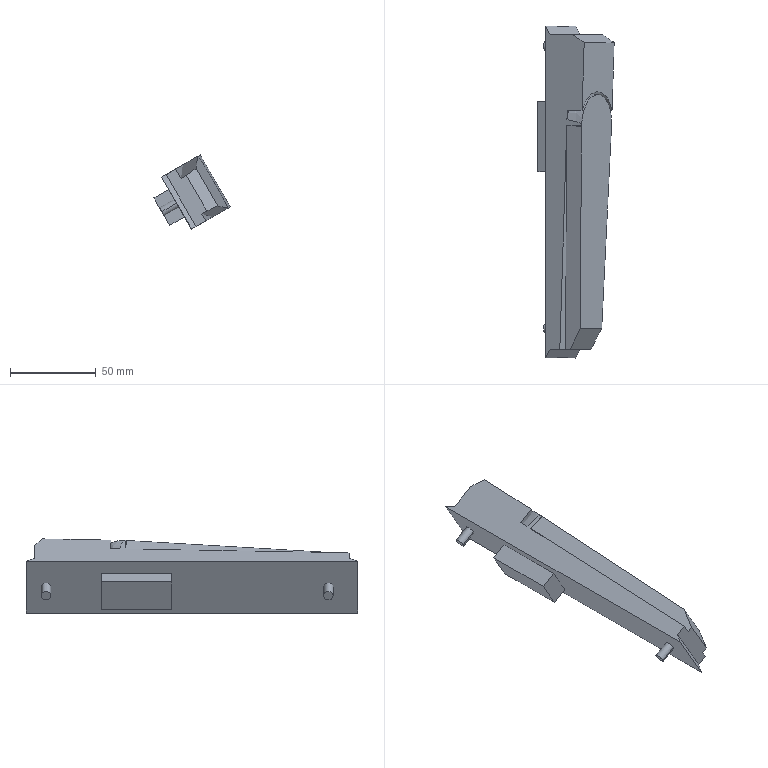Component | SolidWorks | FrontDoorAssembly-1_MS829-1 | 1 solid | 33 faces | box 44.55 x 194 x 43.31 mm | volume 146301 mm3 | plane 24 | cylinder 5 | cone 4 | commonest cylinder face diameters 5.5 x4 35 x1 | material Malleable Cast Iron
STEP:
#1=CARTESIAN_POINT('',(-2.241,37.207,42.755));
#2=VERTEX_POINT('',#1);
#3=CARTESIAN_POINT('',(-2.6,36.76,43.343));
#4=VERTEX_POINT('',#3);
#5=CARTESIAN_POINT('',(-2.265,36.453,42.741));
#6=DIRECTION('',(0.8655,-0.03589,0.4997));
#7=DIRECTION('',(0.03108,0.9994,0.01795));
#8=AXIS2_PLACEMENT_3D('',#5,#6,#7);
#9=CIRCLE('',#8,0.7544);
#10=EDGE_CURVE('',#2,#4,#9,.T.);
#11=ORIENTED_EDGE('',*,*,#10,.F.);
#12=CARTESIAN_POINT('',(-1.9,37.2,42.952));
#13=VERTEX_POINT('',#12);
#14=CARTESIAN_POINT('',(-1.9,37.2,42.952));
#15=DIRECTION('',(0.8659,-0.01845,0.4999));
#16=VECTOR('',#15,39.37);
#17=LINE('',#14,#16);
#18=EDGE_CURVE('',#2,#13,#17,.T.);
#19=ORIENTED_EDGE('',*,*,#18,.T.);
#20=CARTESIAN_POINT('',(-2.258,36.763,43.541));
#21=VERTEX_POINT('',#20);
#22=CARTESIAN_POINT('',(-1.924,36.439,42.938));
#23=DIRECTION('',(0.8655,-0.03589,0.4997));
#24=DIRECTION('',(0.03108,0.9994,0.01795));
#25=AXIS2_PLACEMENT_3D('',#22,#23,#24);
#26=CIRCLE('',#25,0.7613);
#27=EDGE_CURVE('',#13,#21,#26,.T.);
#28=ORIENTED_EDGE('',*,*,#27,.T.);
#29=CARTESIAN_POINT('',(-2.258,36.763,43.541));
#30=CARTESIAN_POINT('',(-2.372,36.762,43.475));
#31=CARTESIAN_POINT('',(-2.486,36.761,43.409));
#32=CARTESIAN_POINT('',(-2.6,36.76,43.343));
#33=B_SPLINE_CURVE_WITH_KNOTS('',3,(#29,#30,#31,#32),.UNSPECIFIED.,.F.,.F.,(4,4),(0.03013,0.04013),.UNSPECIFIED.);
#34=EDGE_CURVE('',#21,#4,#33,.T.);
#35=ORIENTED_EDGE('',*,*,#34,.T.);
#36=EDGE_LOOP('',(#11,#19,#28,#35));
#37=FACE_OUTER_BOUND('',#36,.T.);
#38=CARTESIAN_POINT('',(-1.924,36.439,42.938));
#39=DIRECTION('',(0.8655,-0.03589,0.4997));
#40=DIRECTION('',(0.03108,0.9994,0.01795));
#41=AXIS2_PLACEMENT_3D('',#38,#39,#40);
#42=CONICAL_SURFACE('',#41,0.7613,0.01745);
#43=ADVANCED_FACE('',(#37),#42,.F.);
#44=CARTESIAN_POINT('',(-2.268,36.439,43.535));
#45=VERTEX_POINT('',#44);
#46=CARTESIAN_POINT('',(-1.902,37.128,42.95));
#47=VERTEX_POINT('',#46);
#48=CARTESIAN_POINT('',(-1.924,36.439,42.938));
#49=DIRECTION('',(-0.8655,0.03589,-0.4997));
#50=DIRECTION('',(0.03108,0.9994,0.01795));
#51=AXIS2_PLACEMENT_3D('',#48,#49,#50);
#52=CIRCLE('',#51,0.689);
#53=EDGE_CURVE('',#45,#47,#52,.T.);
#54=ORIENTED_EDGE('',*,*,#53,.T.);
#55=CARTESIAN_POINT('',(-2.243,37.149,42.754));
#56=VERTEX_POINT('',#55);
#57=CARTESIAN_POINT('',(-1.902,37.128,42.95));
#58=DIRECTION('',(-0.8648,0.05333,-0.4993));
#59=VECTOR('',#58,39.37);
#60=LINE('',#57,#59);
#61=EDGE_CURVE('',#47,#56,#60,.T.);
#62=ORIENTED_EDGE('',*,*,#61,.T.);
#63=CARTESIAN_POINT('',(-2.606,36.551,43.34));
#64=VERTEX_POINT('',#63);
#65=CARTESIAN_POINT('',(-2.265,36.453,42.741));
#66=DIRECTION('',(-0.8655,0.03589,-0.4997));
#67=DIRECTION('',(0.03108,0.9994,0.01795));
#68=AXIS2_PLACEMENT_3D('',#65,#66,#67);
#69=CIRCLE('',#68,0.6958);
#70=EDGE_CURVE('',#64,#56,#69,.T.);
#71=ORIENTED_EDGE('',*,*,#70,.F.);
#72=CARTESIAN_POINT('',(-2.606,36.551,43.34));
#73=CARTESIAN_POINT('',(-2.577,36.545,43.357));
#74=CARTESIAN_POINT('',(-2.547,36.539,43.374));
#75=CARTESIAN_POINT('',(-2.489,36.527,43.408));
#76=CARTESIAN_POINT('',(-2.459,36.521,43.425));
#77=CARTESIAN_POINT('',(-2.416,36.51,43.45));
#78=CARTESIAN_POINT('',(-2.401,36.506,43.458));
#79=CARTESIAN_POINT('',(-2.372,36.498,43.475));
#80=CARTESIAN_POINT('',(-2.358,36.493,43.483));
#81=CARTESIAN_POINT('',(-2.329,36.483,43.5));
#82=CARTESIAN_POINT('',(-2.315,36.478,43.508));
#83=CARTESIAN_POINT('',(-2.294,36.468,43.52));
#84=CARTESIAN_POINT('',(-2.288,36.464,43.524));
#85=CARTESIAN_POINT('',(-2.278,36.457,43.529));
#86=CARTESIAN_POINT('',(-2.275,36.454,43.531));
#87=CARTESIAN_POINT('',(-2.272,36.449,43.533));
#88=CARTESIAN_POINT('',(-2.27,36.447,43.534));
#89=CARTESIAN_POINT('',(-2.269,36.443,43.534));
#90=CARTESIAN_POINT('',(-2.268,36.441,43.535));
#91=CARTESIAN_POINT('',(-2.268,36.439,43.535));
#92=B_SPLINE_CURVE_WITH_KNOTS('',3,(#72,#73,#74,#75,#76,#77,#78,#79,#80,#81,#82,#83,#84,#85,#86,#87,#88,#89,#90,#91),.UNSPECIFIED.,.F.,.F.,(4,2,2,2,2,2,2,2,2,4),(0.03208,0.0347,0.03732,0.03863,0.03994,0.04125,0.04191,0.04223,0.0424,0.04256),.UNSPECIFIED.);
#93=EDGE_CURVE('',#64,#45,#92,.T.);
#94=ORIENTED_EDGE('',*,*,#93,.T.);
#95=EDGE_LOOP('',(#54,#62,#71,#94));
#96=FACE_OUTER_BOUND('',#95,.T.);
#97=CARTESIAN_POINT('',(-1.924,36.439,42.938));
#98=DIRECTION('',(-0.8655,0.03589,-0.4997));
#99=DIRECTION('',(0.03108,0.9994,0.01795));
#100=AXIS2_PLACEMENT_3D('',#97,#98,#99);
#101=CONICAL_SURFACE('',#100,0.689,0.01745);
#102=ADVANCED_FACE('',(#96),#101,.T.);
#103=CARTESIAN_POINT('',(-3.093,31.642,42.263));
#104=VERTEX_POINT('',#103);
#105=CARTESIAN_POINT('',(-3.093,31.859,42.263));
#106=VERTEX_POINT('',#105);
#107=CARTESIAN_POINT('',(-3.093,31.75,42.263));
#108=DIRECTION('',(-0.866,-0.,-0.5));
#109=DIRECTION('',(0.,-1.,0.));
#110=AXIS2_PLACEMENT_3D('',#107,#108,#109);
#111=CIRCLE('',#110,0.1083);
#112=EDGE_CURVE('',#104,#106,#111,.T.);
#113=ORIENTED_EDGE('',*,*,#112,.F.);
#114=CARTESIAN_POINT('',(-2.752,31.642,42.46));
#115=VERTEX_POINT('',#114);
#116=CARTESIAN_POINT('',(-3.093,31.642,42.263));
#117=DIRECTION('',(0.866,0.,0.5));
#118=VECTOR('',#117,39.37);
#119=LINE('',#116,#118);
#120=EDGE_CURVE('',#104,#115,#119,.T.);
#121=ORIENTED_EDGE('',*,*,#120,.T.);
#122=CARTESIAN_POINT('',(-2.752,31.859,42.46));
#123=VERTEX_POINT('',#122);
#124=CARTESIAN_POINT('',(-2.752,31.75,42.46));
#125=DIRECTION('',(-0.866,-0.,-0.5));
#126=DIRECTION('',(-0.,1.,0.));
#127=AXIS2_PLACEMENT_3D('',#124,#125,#126);
#128=CIRCLE('',#127,0.1083);
#129=EDGE_CURVE('',#115,#123,#128,.T.);
#130=ORIENTED_EDGE('',*,*,#129,.T.);
#131=CARTESIAN_POINT('',(-3.093,31.859,42.263));
#132=DIRECTION('',(0.866,0.,0.5));
#133=VECTOR('',#132,39.37);
#134=LINE('',#131,#133);
#135=EDGE_CURVE('',#106,#123,#134,.T.);
#136=ORIENTED_EDGE('',*,*,#135,.F.);
#137=EDGE_LOOP('',(#113,#121,#130,#136));
#138=FACE_OUTER_BOUND('',#137,.T.);
#139=CARTESIAN_POINT('',(-3.093,31.75,42.263));
#140=DIRECTION('',(0.866,0.,0.5));
#141=DIRECTION('',(-0.,1.,0.));
#142=AXIS2_PLACEMENT_3D('',#139,#140,#141);
#143=CYLINDRICAL_SURFACE('',#142,0.1083);
#144=ADVANCED_FACE('',(#138),#143,.T.);
#145=CARTESIAN_POINT('',(-3.093,38.138,42.263));
#146=VERTEX_POINT('',#145);
#147=CARTESIAN_POINT('',(-3.093,38.355,42.263));
#148=VERTEX_POINT('',#147);
#149=CARTESIAN_POINT('',(-3.093,38.246,42.263));
#150=DIRECTION('',(-0.866,-0.,-0.5));
#151=DIRECTION('',(0.,-1.,0.));
#152=AXIS2_PLACEMENT_3D('',#149,#150,#151);
#153=CIRCLE('',#152,0.1083);
#154=EDGE_CURVE('',#146,#148,#153,.T.);
#155=ORIENTED_EDGE('',*,*,#154,.F.);
#156=CARTESIAN_POINT('',(-2.752,38.138,42.46));
#157=VERTEX_POINT('',#156);
#158=CARTESIAN_POINT('',(-3.093,38.138,42.263));
#159=DIRECTION('',(0.866,0.,0.5));
#160=VECTOR('',#159,39.37);
#161=LINE('',#158,#160);
#162=EDGE_CURVE('',#146,#157,#161,.T.);
#163=ORIENTED_EDGE('',*,*,#162,.T.);
#164=CARTESIAN_POINT('',(-2.752,38.355,42.46));
#165=VERTEX_POINT('',#164);
#166=CARTESIAN_POINT('',(-2.752,38.246,42.46));
#167=DIRECTION('',(-0.866,-0.,-0.5));
#168=DIRECTION('',(-0.,1.,0.));
#169=AXIS2_PLACEMENT_3D('',#166,#167,#168);
#170=CIRCLE('',#169,0.1083);
#171=EDGE_CURVE('',#157,#165,#170,.T.);
#172=ORIENTED_EDGE('',*,*,#171,.T.);
#173=CARTESIAN_POINT('',(-3.093,38.355,42.263));
#174=DIRECTION('',(0.866,0.,0.5));
#175=VECTOR('',#174,39.37);
#176=LINE('',#173,#175);
#177=EDGE_CURVE('',#148,#165,#176,.T.);
#178=ORIENTED_EDGE('',*,*,#177,.F.);
#179=EDGE_LOOP('',(#155,#163,#172,#178));
#180=FACE_OUTER_BOUND('',#179,.T.);
#181=CARTESIAN_POINT('',(-3.093,38.246,42.263));
#182=DIRECTION('',(0.866,0.,0.5));
#183=DIRECTION('',(-0.,1.,0.));
#184=AXIS2_PLACEMENT_3D('',#181,#182,#183);
#185=CYLINDRICAL_SURFACE('',#184,0.1083);
#186=ADVANCED_FACE('',(#180),#185,.T.);
#187=CARTESIAN_POINT('',(-2.27,36.4,43.534));
#188=VERTEX_POINT('',#187);
#189=CARTESIAN_POINT('',(-2.21,38.326,43.569));
#190=DIRECTION('',(0.03108,0.9994,0.01795));
#191=VECTOR('',#190,39.37);
#192=LINE('',#189,#191);
#193=EDGE_CURVE('',#188,#45,#192,.T.);
#194=ORIENTED_EDGE('',*,*,#193,.F.);
#195=CARTESIAN_POINT('',(-2.269,36.406,43.533));
#196=VERTEX_POINT('',#195);
#197=CARTESIAN_POINT('',(-2.161,37.603,43.433));
#198=DIRECTION('',(0.08924,0.9925,-0.08327));
#199=VECTOR('',#198,39.37);
#200=LINE('',#197,#199);
#201=EDGE_CURVE('',#188,#196,#200,.T.);
#202=ORIENTED_EDGE('',*,*,#201,.T.);
#203=CARTESIAN_POINT('',(-2.303,31.749,43.258));
#204=VERTEX_POINT('',#203);
#205=CARTESIAN_POINT('',(-2.262,37.39,43.592));
#206=DIRECTION('',(-0.007358,-0.9982,-0.05896));
#207=VECTOR('',#206,39.37);
#208=LINE('',#205,#207);
#209=EDGE_CURVE('',#196,#204,#208,.T.);
#210=ORIENTED_EDGE('',*,*,#209,.T.);
#211=CARTESIAN_POINT('',(-1.807,31.749,42.399));
#212=VERTEX_POINT('',#211);
#213=CARTESIAN_POINT('',(-1.725,31.749,42.257));
#214=DIRECTION('',(-0.5,-0.,0.866));
#215=VECTOR('',#214,39.37);
#216=LINE('',#213,#215);
#217=EDGE_CURVE('',#212,#204,#216,.T.);
#218=ORIENTED_EDGE('',*,*,#217,.F.);
#219=CARTESIAN_POINT('',(-1.582,36.391,42.342));
#220=VERTEX_POINT('',#219);
#221=CARTESIAN_POINT('',(-1.53,37.457,42.329));
#222=DIRECTION('',(-0.04852,-0.9987,0.0123));
#223=VECTOR('',#222,39.37);
#224=LINE('',#221,#223);
#225=EDGE_CURVE('',#220,#212,#224,.T.);
#226=ORIENTED_EDGE('',*,*,#225,.F.);
#227=CARTESIAN_POINT('',(-1.579,36.439,42.341));
#228=VERTEX_POINT('',#227);
#229=CARTESIAN_POINT('',(-1.924,36.439,42.938));
#230=DIRECTION('',(0.8655,-0.03589,0.4997));
#231=DIRECTION('',(0.03108,0.9994,0.01795));
#232=AXIS2_PLACEMENT_3D('',#229,#230,#231);
#233=CIRCLE('',#232,0.689);
#234=EDGE_CURVE('',#220,#228,#233,.T.);
#235=ORIENTED_EDGE('',*,*,#234,.T.);
#236=CARTESIAN_POINT('',(-1.924,36.439,42.938));
#237=DIRECTION('',(-0.8655,0.03589,-0.4997));
#238=DIRECTION('',(0.03108,0.9994,0.01795));
#239=AXIS2_PLACEMENT_3D('',#236,#237,#238);
#240=CIRCLE('',#239,0.689);
#241=EDGE_CURVE('',#47,#228,#240,.T.);
#242=ORIENTED_EDGE('',*,*,#241,.F.);
#243=ORIENTED_EDGE('',*,*,#53,.F.);
#244=EDGE_LOOP('',(#194,#202,#210,#218,#226,#235,#242,#243));
#245=FACE_OUTER_BOUND('',#244,.T.);
#246=CARTESIAN_POINT('',(-1.521,38.326,42.375));
#247=DIRECTION('',(0.8655,-0.03589,0.4997));
#248=DIRECTION('',(0.03108,0.9994,0.01795));
#249=AXIS2_PLACEMENT_3D('',#246,#247,#248);
#250=PLANE('',#249);
#251=ADVANCED_FACE('',(#245),#250,.T.);
#252=CARTESIAN_POINT('',(-2.77,31.266,43.245));
#253=VERTEX_POINT('',#252);
#254=CARTESIAN_POINT('',(-2.61,36.414,43.337));
#255=VERTEX_POINT('',#254);
#256=CARTESIAN_POINT('',(-2.577,37.472,43.356));
#257=DIRECTION('',(0.03108,0.9994,0.01795));
#258=VECTOR('',#257,39.37);
#259=LINE('',#256,#258);
#260=EDGE_CURVE('',#253,#255,#259,.T.);
#261=ORIENTED_EDGE('',*,*,#260,.T.);
#262=CARTESIAN_POINT('',(-1.089,36.351,44.215));
#263=DIRECTION('',(0.8655,-0.03589,0.4997));
#264=VECTOR('',#263,39.37);
#265=LINE('',#262,#264);
#266=EDGE_CURVE('',#255,#188,#265,.T.);
#267=ORIENTED_EDGE('',*,*,#266,.T.);
#268=ORIENTED_EDGE('',*,*,#193,.T.);
#269=ORIENTED_EDGE('',*,*,#93,.F.);
#270=CARTESIAN_POINT('',(-2.577,37.472,43.356));
#271=DIRECTION('',(0.03108,0.9994,0.01795));
#272=VECTOR('',#271,39.37);
#273=LINE('',#270,#272);
#274=EDGE_CURVE('',#64,#4,#273,.T.);
#275=ORIENTED_EDGE('',*,*,#274,.T.);
#276=ORIENTED_EDGE('',*,*,#34,.F.);
#277=CARTESIAN_POINT('',(-2.21,38.326,43.569));
#278=VERTEX_POINT('',#277);
#279=CARTESIAN_POINT('',(-2.21,38.326,43.569));
#280=DIRECTION('',(0.03108,0.9994,0.01795));
#281=VECTOR('',#280,39.37);
#282=LINE('',#279,#281);
#283=EDGE_CURVE('',#21,#278,#282,.T.);
#284=ORIENTED_EDGE('',*,*,#283,.T.);
#285=CARTESIAN_POINT('',(-2.476,38.51,43.415));
#286=VERTEX_POINT('',#285);
#287=CARTESIAN_POINT('',(-2.476,38.51,43.415));
#288=DIRECTION('',(-0.7426,0.5145,-0.4287));
#289=VECTOR('',#288,39.37);
#290=LINE('',#287,#289);
#291=EDGE_CURVE('',#278,#286,#290,.T.);
#292=ORIENTED_EDGE('',*,*,#291,.T.);
#293=CARTESIAN_POINT('',(-2.994,38.51,43.116));
#294=VERTEX_POINT('',#293);
#295=CARTESIAN_POINT('',(-2.994,38.51,43.116));
#296=DIRECTION('',(-0.866,-0.,-0.5));
#297=VECTOR('',#296,39.37);
#298=LINE('',#295,#297);
#299=EDGE_CURVE('',#286,#294,#298,.T.);
#300=ORIENTED_EDGE('',*,*,#299,.T.);
#301=CARTESIAN_POINT('',(-3.096,38.707,43.057));
#302=VERTEX_POINT('',#301);
#303=CARTESIAN_POINT('',(-3.096,38.707,43.057));
#304=DIRECTION('',(-0.4456,0.8575,-0.2572));
#305=VECTOR('',#304,39.37);
#306=LINE('',#303,#305);
#307=EDGE_CURVE('',#294,#302,#306,.T.);
#308=ORIENTED_EDGE('',*,*,#307,.T.);
#309=CARTESIAN_POINT('',(-3.096,31.069,43.057));
#310=VERTEX_POINT('',#309);
#311=CARTESIAN_POINT('',(-3.096,38.707,43.057));
#312=DIRECTION('',(0.,-1.,-0.));
#313=VECTOR('',#312,39.37);
#314=LINE('',#311,#313);
#315=EDGE_CURVE('',#302,#310,#314,.T.);
#316=ORIENTED_EDGE('',*,*,#315,.T.);
#317=CARTESIAN_POINT('',(-2.994,31.266,43.116));
#318=VERTEX_POINT('',#317);
#319=CARTESIAN_POINT('',(-3.096,31.069,43.057));
#320=DIRECTION('',(0.4456,0.8575,0.2572));
#321=VECTOR('',#320,39.37);
#322=LINE('',#319,#321);
#323=EDGE_CURVE('',#310,#318,#322,.T.);
#324=ORIENTED_EDGE('',*,*,#323,.T.);
#325=CARTESIAN_POINT('',(-2.994,31.266,43.116));
#326=DIRECTION('',(0.866,0.,0.5));
#327=VECTOR('',#326,39.37);
#328=LINE('',#325,#327);
#329=EDGE_CURVE('',#318,#253,#328,.T.);
#330=ORIENTED_EDGE('',*,*,#329,.T.);
#331=EDGE_LOOP('',(#261,#267,#268,#269,#275,#276,#284,#292,#300,#308,#316,#324,#330));
#332=FACE_OUTER_BOUND('',#331,.T.);
#333=CARTESIAN_POINT('',(-1.056,37.409,44.234));
#334=DIRECTION('',(-0.5,-0.,0.866));
#335=DIRECTION('',(0.866,0.,0.5));
#336=AXIS2_PLACEMENT_3D('',#333,#334,#335);
#337=PLANE('',#336);
#338=ADVANCED_FACE('',(#332),#337,.T.);
#339=CARTESIAN_POINT('',(-1.92,36.453,42.145));
#340=VERTEX_POINT('',#339);
#341=CARTESIAN_POINT('',(-1.92,36.453,42.145));
#342=DIRECTION('',(0.8655,-0.03589,0.4997));
#343=VECTOR('',#342,39.37);
#344=LINE('',#341,#343);
#345=EDGE_CURVE('',#340,#228,#344,.T.);
#346=ORIENTED_EDGE('',*,*,#345,.F.);
#347=CARTESIAN_POINT('',(-2.081,31.266,42.051));
#348=VERTEX_POINT('',#347);
#349=CARTESIAN_POINT('',(-1.888,37.472,42.163));
#350=DIRECTION('',(0.03108,0.9994,0.01795));
#351=VECTOR('',#350,39.37);
#352=LINE('',#349,#351);
#353=EDGE_CURVE('',#348,#340,#352,.T.);
#354=ORIENTED_EDGE('',*,*,#353,.F.);
#355=CARTESIAN_POINT('',(-2.305,31.266,41.922));
#356=VERTEX_POINT('',#355);
#357=CARTESIAN_POINT('',(-2.305,31.266,41.922));
#358=DIRECTION('',(0.866,0.,0.5));
#359=VECTOR('',#358,39.37);
#360=LINE('',#357,#359);
#361=EDGE_CURVE('',#356,#348,#360,.T.);
#362=ORIENTED_EDGE('',*,*,#361,.F.);
#363=CARTESIAN_POINT('',(-2.407,31.069,41.863));
#364=VERTEX_POINT('',#363);
#365=CARTESIAN_POINT('',(-2.407,31.069,41.863));
#366=DIRECTION('',(0.4456,0.8575,0.2572));
#367=VECTOR('',#366,39.37);
#368=LINE('',#365,#367);
#369=EDGE_CURVE('',#364,#356,#368,.T.);
#370=ORIENTED_EDGE('',*,*,#369,.F.);
#371=CARTESIAN_POINT('',(-2.407,38.707,41.863));
#372=VERTEX_POINT('',#371);
#373=CARTESIAN_POINT('',(-2.407,38.707,41.863));
#374=DIRECTION('',(0.,-1.,-0.));
#375=VECTOR('',#374,39.37);
#376=LINE('',#373,#375);
#377=EDGE_CURVE('',#372,#364,#376,.T.);
#378=ORIENTED_EDGE('',*,*,#377,.F.);
#379=CARTESIAN_POINT('',(-2.305,38.51,41.922));
#380=VERTEX_POINT('',#379);
#381=CARTESIAN_POINT('',(-2.407,38.707,41.863));
#382=DIRECTION('',(-0.4456,0.8575,-0.2572));
#383=VECTOR('',#382,39.37);
#384=LINE('',#381,#383);
#385=EDGE_CURVE('',#380,#372,#384,.T.);
#386=ORIENTED_EDGE('',*,*,#385,.F.);
#387=CARTESIAN_POINT('',(-1.787,38.51,42.222));
#388=VERTEX_POINT('',#387);
#389=CARTESIAN_POINT('',(-2.305,38.51,41.922));
#390=DIRECTION('',(-0.866,-0.,-0.5));
#391=VECTOR('',#390,39.37);
#392=LINE('',#389,#391);
#393=EDGE_CURVE('',#388,#380,#392,.T.);
#394=ORIENTED_EDGE('',*,*,#393,.F.);
#395=CARTESIAN_POINT('',(-1.521,38.326,42.375));
#396=VERTEX_POINT('',#395);
#397=CARTESIAN_POINT('',(-1.787,38.51,42.222));
#398=DIRECTION('',(-0.7426,0.5145,-0.4287));
#399=VECTOR('',#398,39.37);
#400=LINE('',#397,#399);
#401=EDGE_CURVE('',#396,#388,#400,.T.);
#402=ORIENTED_EDGE('',*,*,#401,.F.);
#403=CARTESIAN_POINT('',(-1.569,36.763,42.347));
#404=VERTEX_POINT('',#403);
#405=CARTESIAN_POINT('',(-1.521,38.326,42.375));
#406=DIRECTION('',(0.03108,0.9994,0.01795));
#407=VECTOR('',#406,39.37);
#408=LINE('',#405,#407);
#409=EDGE_CURVE('',#404,#396,#408,.T.);
#410=ORIENTED_EDGE('',*,*,#409,.F.);
#411=CARTESIAN_POINT('',(-1.911,36.76,42.15));
#412=VERTEX_POINT('',#411);
#413=CARTESIAN_POINT('',(-1.569,36.763,42.347));
#414=CARTESIAN_POINT('',(-1.683,36.762,42.281));
#415=CARTESIAN_POINT('',(-1.797,36.761,42.216));
#416=CARTESIAN_POINT('',(-1.911,36.76,42.15));
#417=B_SPLINE_CURVE_WITH_KNOTS('',3,(#413,#414,#415,#416),.UNSPECIFIED.,.F.,.F.,(4,4),(0.03013,0.04013),.UNSPECIFIED.);
#418=EDGE_CURVE('',#404,#412,#417,.T.);
#419=ORIENTED_EDGE('',*,*,#418,.T.);
#420=CARTESIAN_POINT('',(-1.917,36.551,42.146));
#421=VERTEX_POINT('',#420);
#422=CARTESIAN_POINT('',(-1.888,37.472,42.163));
#423=DIRECTION('',(0.03108,0.9994,0.01795));
#424=VECTOR('',#423,39.37);
#425=LINE('',#422,#424);
#426=EDGE_CURVE('',#421,#412,#425,.T.);
#427=ORIENTED_EDGE('',*,*,#426,.F.);
#428=CARTESIAN_POINT('',(-1.917,36.551,42.146));
#429=CARTESIAN_POINT('',(-1.888,36.545,42.163));
#430=CARTESIAN_POINT('',(-1.858,36.539,42.18));
#431=CARTESIAN_POINT('',(-1.8,36.527,42.214));
#432=CARTESIAN_POINT('',(-1.77,36.521,42.231));
#433=CARTESIAN_POINT('',(-1.727,36.51,42.256));
#434=CARTESIAN_POINT('',(-1.712,36.506,42.265));
#435=CARTESIAN_POINT('',(-1.683,36.498,42.282));
#436=CARTESIAN_POINT('',(-1.669,36.493,42.29));
#437=CARTESIAN_POINT('',(-1.64,36.483,42.306));
#438=CARTESIAN_POINT('',(-1.626,36.478,42.315));
#439=CARTESIAN_POINT('',(-1.605,36.468,42.326));
#440=CARTESIAN_POINT('',(-1.599,36.464,42.33));
#441=CARTESIAN_POINT('',(-1.589,36.457,42.336));
#442=CARTESIAN_POINT('',(-1.586,36.454,42.337));
#443=CARTESIAN_POINT('',(-1.583,36.449,42.34));
#444=CARTESIAN_POINT('',(-1.581,36.447,42.34));
#445=CARTESIAN_POINT('',(-1.58,36.443,42.341));
#446=CARTESIAN_POINT('',(-1.579,36.441,42.341));
#447=CARTESIAN_POINT('',(-1.579,36.439,42.341));
#448=B_SPLINE_CURVE_WITH_KNOTS('',3,(#428,#429,#430,#431,#432,#433,#434,#435,#436,#437,#438,#439,#440,#441,#442,#443,#444,#445,#446,#447),.UNSPECIFIED.,.F.,.F.,(4,2,2,2,2,2,2,2,2,4),(0.03208,0.0347,0.03732,0.03863,0.03994,0.04125,0.04191,0.04223,0.0424,0.04256),.UNSPECIFIED.);
#449=EDGE_CURVE('',#421,#228,#448,.T.);
#450=ORIENTED_EDGE('',*,*,#449,.T.);
#451=EDGE_LOOP('',(#346,#354,#362,#370,#378,#386,#394,#402,#410,#419,#427,#450));
#452=FACE_OUTER_BOUND('',#451,.T.);
#453=CARTESIAN_POINT('',(-0.3675,37.409,43.041));
#454=DIRECTION('',(-0.5,-0.,0.866));
#455=DIRECTION('',(0.866,0.,0.5));
#456=AXIS2_PLACEMENT_3D('',#453,#454,#455);
#457=PLANE('',#456);
#458=ADVANCED_FACE('',(#452),#457,.F.);
#459=ORIENTED_EDGE('',*,*,#217,.T.);
#460=CARTESIAN_POINT('',(-2.53,31.266,43.1));
#461=VERTEX_POINT('',#460);
#462=CARTESIAN_POINT('',(-2.55,31.225,43.087));
#463=DIRECTION('',(-0.408,-0.8677,-0.284));
#464=VECTOR('',#463,39.37);
#465=LINE('',#462,#464);
#466=EDGE_CURVE('',#204,#461,#465,.T.);
#467=ORIENTED_EDGE('',*,*,#466,.T.);
#468=CARTESIAN_POINT('',(-2.055,31.266,42.276));
#469=VERTEX_POINT('',#468);
#470=CARTESIAN_POINT('',(-1.964,31.266,42.119));
#471=DIRECTION('',(-0.5,-0.,0.866));
#472=VECTOR('',#471,39.37);
#473=LINE('',#470,#472);
#474=EDGE_CURVE('',#469,#461,#473,.T.);
#475=ORIENTED_EDGE('',*,*,#474,.F.);
#476=CARTESIAN_POINT('',(-2.052,31.271,42.277));
#477=DIRECTION('',(-0.4446,-0.868,-0.221));
#478=VECTOR('',#477,39.37);
#479=LINE('',#476,#478);
#480=EDGE_CURVE('',#212,#469,#479,.T.);
#481=ORIENTED_EDGE('',*,*,#480,.F.);
#482=EDGE_LOOP('',(#459,#467,#475,#481));
#483=FACE_OUTER_BOUND('',#482,.T.);
#484=CARTESIAN_POINT('',(-1.964,31.266,42.119));
#485=DIRECTION('',(0.7521,-0.4958,0.4342));
#486=DIRECTION('',(0.4293,0.8685,0.2479));
#487=AXIS2_PLACEMENT_3D('',#484,#485,#486);
#488=PLANE('',#487);
#489=ADVANCED_FACE('',(#483),#488,.T.);
#490=CARTESIAN_POINT('',(-2.172,31.266,42.209));
#491=VERTEX_POINT('',#490);
#492=CARTESIAN_POINT('',(-2.396,31.266,42.08));
#493=DIRECTION('',(-0.8667,-0.,-0.4989));
#494=VECTOR('',#493,39.37);
#495=LINE('',#492,#494);
#496=EDGE_CURVE('',#469,#491,#495,.T.);
#497=ORIENTED_EDGE('',*,*,#496,.F.);
#498=ORIENTED_EDGE('',*,*,#474,.T.);
#499=CARTESIAN_POINT('',(-2.648,31.266,43.032));
#500=VERTEX_POINT('',#499);
#501=CARTESIAN_POINT('',(-2.873,31.266,42.902));
#502=DIRECTION('',(-0.8652,-0.,-0.5015));
#503=VECTOR('',#502,39.37);
#504=LINE('',#501,#503);
#505=EDGE_CURVE('',#461,#500,#504,.T.);
#506=ORIENTED_EDGE('',*,*,#505,.T.);
#507=CARTESIAN_POINT('',(-2.081,31.266,42.051));
#508=DIRECTION('',(-0.5,-0.,0.866));
#509=VECTOR('',#508,39.37);
#510=LINE('',#507,#509);
#511=EDGE_CURVE('',#500,#253,#510,.T.);
#512=ORIENTED_EDGE('',*,*,#511,.T.);
#513=ORIENTED_EDGE('',*,*,#329,.F.);
#514=CARTESIAN_POINT('',(-2.305,31.266,41.922));
#515=DIRECTION('',(-0.5,-0.,0.866));
#516=VECTOR('',#515,39.37);
#517=LINE('',#514,#516);
#518=EDGE_CURVE('',#356,#318,#517,.T.);
#519=ORIENTED_EDGE('',*,*,#518,.F.);
#520=ORIENTED_EDGE('',*,*,#361,.T.);
#521=CARTESIAN_POINT('',(-2.081,31.266,42.051));
#522=DIRECTION('',(-0.5,-0.,0.866));
#523=VECTOR('',#522,39.37);
#524=LINE('',#521,#523);
#525=EDGE_CURVE('',#348,#491,#524,.T.);
#526=ORIENTED_EDGE('',*,*,#525,.T.);
#527=EDGE_LOOP('',(#497,#498,#506,#512,#513,#519,#520,#526));
#528=FACE_OUTER_BOUND('',#527,.T.);
#529=CARTESIAN_POINT('',(-2.305,31.266,41.922));
#530=DIRECTION('',(0.,-1.,-0.));
#531=DIRECTION('',(0.5,0.,-0.866));
#532=AXIS2_PLACEMENT_3D('',#529,#530,#531);
#533=PLANE('',#532);
#534=ADVANCED_FACE('',(#528),#533,.T.);
#535=CARTESIAN_POINT('',(-2.752,38.246,42.46));
#536=DIRECTION('',(-0.866,-0.,-0.5));
#537=DIRECTION('',(-0.,1.,0.));
#538=AXIS2_PLACEMENT_3D('',#535,#536,#537);
#539=CIRCLE('',#538,0.1083);
#540=EDGE_CURVE('',#165,#157,#539,.T.);
#541=ORIENTED_EDGE('',*,*,#540,.F.);
#542=ORIENTED_EDGE('',*,*,#171,.F.);
#543=EDGE_LOOP('',(#541,#542));
#544=FACE_BOUND('',#543,.T.);
#545=ORIENTED_EDGE('',*,*,#377,.T.);
#546=CARTESIAN_POINT('',(-3.096,31.069,43.057));
#547=DIRECTION('',(0.5,0.,-0.866));
#548=VECTOR('',#547,39.37);
#549=LINE('',#546,#548);
#550=EDGE_CURVE('',#310,#364,#549,.T.);
#551=ORIENTED_EDGE('',*,*,#550,.F.);
#552=ORIENTED_EDGE('',*,*,#315,.F.);
#553=CARTESIAN_POINT('',(-3.096,38.707,43.057));
#554=DIRECTION('',(0.5,0.,-0.866));
#555=VECTOR('',#554,39.37);
#556=LINE('',#553,#555);
#557=EDGE_CURVE('',#302,#372,#556,.T.);
#558=ORIENTED_EDGE('',*,*,#557,.T.);
#559=EDGE_LOOP('',(#545,#551,#552,#558));
#560=FACE_OUTER_BOUND('',#559,.T.);
#561=CARTESIAN_POINT('',(-2.57,36.967,42.145));
#562=VERTEX_POINT('',#561);
#563=CARTESIAN_POINT('',(-2.57,35.353,42.145));
#564=VERTEX_POINT('',#563);
#565=CARTESIAN_POINT('',(-2.57,36.967,42.145));
#566=DIRECTION('',(0.,-1.,-0.));
#567=VECTOR('',#566,39.37);
#568=LINE('',#565,#567);
#569=EDGE_CURVE('',#562,#564,#568,.T.);
#570=ORIENTED_EDGE('',*,*,#569,.F.);
#571=CARTESIAN_POINT('',(-2.934,36.967,42.775));
#572=VERTEX_POINT('',#571);
#573=CARTESIAN_POINT('',(-2.57,36.967,42.145));
#574=DIRECTION('',(0.5,0.,-0.866));
#575=VECTOR('',#574,39.37);
#576=LINE('',#573,#575);
#577=EDGE_CURVE('',#572,#562,#576,.T.);
#578=ORIENTED_EDGE('',*,*,#577,.F.);
#579=CARTESIAN_POINT('',(-2.934,35.353,42.775));
#580=VERTEX_POINT('',#579);
#581=CARTESIAN_POINT('',(-2.934,36.967,42.775));
#582=DIRECTION('',(-0.,1.,0.));
#583=VECTOR('',#582,39.37);
#584=LINE('',#581,#583);
#585=EDGE_CURVE('',#580,#572,#584,.T.);
#586=ORIENTED_EDGE('',*,*,#585,.F.);
#587=CARTESIAN_POINT('',(-2.57,35.353,42.145));
#588=DIRECTION('',(-0.5,-0.,0.866));
#589=VECTOR('',#588,39.37);
#590=LINE('',#587,#589);
#591=EDGE_CURVE('',#564,#580,#590,.T.);
#592=ORIENTED_EDGE('',*,*,#591,.F.);
#593=EDGE_LOOP('',(#570,#578,#586,#592));
#594=FACE_BOUND('',#593,.T.);
#595=CARTESIAN_POINT('',(-2.752,31.75,42.46));
#596=DIRECTION('',(-0.866,-0.,-0.5));
#597=DIRECTION('',(0.,1.,-0.));
#598=AXIS2_PLACEMENT_3D('',#595,#596,#597);
#599=CIRCLE('',#598,0.1083);
#600=EDGE_CURVE('',#123,#115,#599,.T.);
#601=ORIENTED_EDGE('',*,*,#600,.F.);
#602=ORIENTED_EDGE('',*,*,#129,.F.);
#603=EDGE_LOOP('',(#601,#602));
#604=FACE_BOUND('',#603,.T.);
#605=CARTESIAN_POINT('',(-3.096,38.707,43.057));
#606=DIRECTION('',(0.866,0.,0.5));
#607=DIRECTION('',(-0.,1.,0.));
#608=AXIS2_PLACEMENT_3D('',#605,#606,#607);
#609=PLANE('',#608);
#610=ADVANCED_FACE('',(#544,#560,#594,#604),#609,.F.);
#611=ORIENTED_EDGE('',*,*,#299,.F.);
#612=CARTESIAN_POINT('',(-1.787,38.51,42.222));
#613=DIRECTION('',(-0.5,-0.,0.866));
#614=VECTOR('',#613,39.37);
#615=LINE('',#612,#614);
#616=EDGE_CURVE('',#388,#286,#615,.T.);
#617=ORIENTED_EDGE('',*,*,#616,.F.);
#618=ORIENTED_EDGE('',*,*,#393,.T.);
#619=CARTESIAN_POINT('',(-2.305,38.51,41.922));
#620=DIRECTION('',(-0.5,-0.,0.866));
#621=VECTOR('',#620,39.37);
#622=LINE('',#619,#621);
#623=EDGE_CURVE('',#380,#294,#622,.T.);
#624=ORIENTED_EDGE('',*,*,#623,.T.);
#625=EDGE_LOOP('',(#611,#617,#618,#624));
#626=FACE_OUTER_BOUND('',#625,.T.);
#627=CARTESIAN_POINT('',(-2.305,38.51,41.922));
#628=DIRECTION('',(-0.,1.,0.));
#629=DIRECTION('',(-0.5,-0.,0.866));
#630=AXIS2_PLACEMENT_3D('',#627,#628,#629);
#631=PLANE('',#630);
#632=ADVANCED_FACE('',(#626),#631,.T.);
#633=ORIENTED_EDGE('',*,*,#291,.F.);
#634=CARTESIAN_POINT('',(-1.521,38.326,42.375));
#635=DIRECTION('',(-0.5,-0.,0.866));
#636=VECTOR('',#635,39.37);
#637=LINE('',#634,#636);
#638=EDGE_CURVE('',#396,#278,#637,.T.);
#639=ORIENTED_EDGE('',*,*,#638,.F.);
#640=ORIENTED_EDGE('',*,*,#401,.T.);
#641=ORIENTED_EDGE('',*,*,#616,.T.);
#642=EDGE_LOOP('',(#633,#639,#640,#641));
#643=FACE_OUTER_BOUND('',#642,.T.);
#644=CARTESIAN_POINT('',(-1.787,38.51,42.222));
#645=DIRECTION('',(0.4456,0.8575,0.2572));
#646=DIRECTION('',(-0.7426,0.5145,-0.4287));
#647=AXIS2_PLACEMENT_3D('',#644,#645,#646);
#648=PLANE('',#647);
#649=ADVANCED_FACE('',(#643),#648,.T.);
#650=CARTESIAN_POINT('',(-1.924,36.439,42.938));
#651=DIRECTION('',(0.8655,-0.03589,0.4997));
#652=DIRECTION('',(0.03108,0.9994,0.01795));
#653=AXIS2_PLACEMENT_3D('',#650,#651,#652);
#654=CIRCLE('',#653,0.7613);
#655=EDGE_CURVE('',#404,#13,#654,.T.);
#656=ORIENTED_EDGE('',*,*,#655,.F.);
#657=ORIENTED_EDGE('',*,*,#409,.T.);
#658=ORIENTED_EDGE('',*,*,#638,.T.);
#659=ORIENTED_EDGE('',*,*,#283,.F.);
#660=ORIENTED_EDGE('',*,*,#27,.F.);
#661=EDGE_LOOP('',(#656,#657,#658,#659,#660));
#662=FACE_OUTER_BOUND('',#661,.T.);
#663=CARTESIAN_POINT('',(-1.521,38.326,42.375));
#664=DIRECTION('',(0.8655,-0.03589,0.4997));
#665=DIRECTION('',(0.03108,0.9994,0.01795));
#666=AXIS2_PLACEMENT_3D('',#663,#664,#665);
#667=PLANE('',#666);
#668=ADVANCED_FACE('',(#662),#667,.T.);
#669=ORIENTED_EDGE('',*,*,#323,.F.);
#670=ORIENTED_EDGE('',*,*,#550,.T.);
#671=ORIENTED_EDGE('',*,*,#369,.T.);
#672=ORIENTED_EDGE('',*,*,#518,.T.);
#673=EDGE_LOOP('',(#669,#670,#671,#672));
#674=FACE_OUTER_BOUND('',#673,.T.);
#675=CARTESIAN_POINT('',(-2.407,31.069,41.863));
#676=DIRECTION('',(0.7426,-0.5145,0.4287));
#677=DIRECTION('',(0.4456,0.8575,0.2572));
#678=AXIS2_PLACEMENT_3D('',#675,#676,#677);
#679=PLANE('',#678);
#680=ADVANCED_FACE('',(#674),#679,.T.);
#681=ORIENTED_EDGE('',*,*,#307,.F.);
#682=ORIENTED_EDGE('',*,*,#623,.F.);
#683=ORIENTED_EDGE('',*,*,#385,.T.);
#684=ORIENTED_EDGE('',*,*,#557,.F.);
#685=EDGE_LOOP('',(#681,#682,#683,#684));
#686=FACE_OUTER_BOUND('',#685,.T.);
#687=CARTESIAN_POINT('',(-2.407,38.707,41.863));
#688=DIRECTION('',(0.7426,0.5145,0.4287));
#689=DIRECTION('',(-0.4456,0.8575,-0.2572));
#690=AXIS2_PLACEMENT_3D('',#687,#688,#689);
#691=PLANE('',#690);
#692=ADVANCED_FACE('',(#686),#691,.T.);
#693=ORIENTED_EDGE('',*,*,#569,.T.);
#694=CARTESIAN_POINT('',(-2.911,35.353,41.948));
#695=VERTEX_POINT('',#694);
#696=CARTESIAN_POINT('',(-2.911,35.353,41.948));
#697=DIRECTION('',(0.866,0.,0.5));
#698=VECTOR('',#697,39.37);
#699=LINE('',#696,#698);
#700=EDGE_CURVE('',#695,#564,#699,.T.);
#701=ORIENTED_EDGE('',*,*,#700,.F.);
#702=CARTESIAN_POINT('',(-2.911,36.967,41.948));
#703=VERTEX_POINT('',#702);
#704=CARTESIAN_POINT('',(-2.911,36.967,41.948));
#705=DIRECTION('',(0.,-1.,-0.));
#706=VECTOR('',#705,39.37);
#707=LINE('',#704,#706);
#708=EDGE_CURVE('',#703,#695,#707,.T.);
#709=ORIENTED_EDGE('',*,*,#708,.F.);
#710=CARTESIAN_POINT('',(-2.911,36.967,41.948));
#711=DIRECTION('',(0.866,0.,0.5));
#712=VECTOR('',#711,39.37);
#713=LINE('',#710,#712);
#714=EDGE_CURVE('',#703,#562,#713,.T.);
#715=ORIENTED_EDGE('',*,*,#714,.T.);
#716=EDGE_LOOP('',(#693,#701,#709,#715));
#717=FACE_OUTER_BOUND('',#716,.T.);
#718=CARTESIAN_POINT('',(-2.911,36.967,41.948));
#719=DIRECTION('',(-0.5,-0.,0.866));
#720=DIRECTION('',(0.,-1.,-0.));
#721=AXIS2_PLACEMENT_3D('',#718,#719,#720);
#722=PLANE('',#721);
#723=ADVANCED_FACE('',(#717),#722,.F.);
#724=ORIENTED_EDGE('',*,*,#591,.T.);
#725=CARTESIAN_POINT('',(-3.275,35.353,42.579));
#726=VERTEX_POINT('',#725);
#727=CARTESIAN_POINT('',(-3.275,35.353,42.579));
#728=DIRECTION('',(0.866,0.,0.5));
#729=VECTOR('',#728,39.37);
#730=LINE('',#727,#729);
#731=EDGE_CURVE('',#726,#580,#730,.T.);
#732=ORIENTED_EDGE('',*,*,#731,.F.);
#733=CARTESIAN_POINT('',(-2.911,35.353,41.948));
#734=DIRECTION('',(-0.5,-0.,0.866));
#735=VECTOR('',#734,39.37);
#736=LINE('',#733,#735);
#737=EDGE_CURVE('',#695,#726,#736,.T.);
#738=ORIENTED_EDGE('',*,*,#737,.F.);
#739=ORIENTED_EDGE('',*,*,#700,.T.);
#740=EDGE_LOOP('',(#724,#732,#738,#739));
#741=FACE_OUTER_BOUND('',#740,.T.);
#742=CARTESIAN_POINT('',(-2.911,35.353,41.948));
#743=DIRECTION('',(-0.,1.,0.));
#744=DIRECTION('',(-0.866,-0.,-0.5));
#745=AXIS2_PLACEMENT_3D('',#742,#743,#744);
#746=PLANE('',#745);
#747=ADVANCED_FACE('',(#741),#746,.F.);
#748=ORIENTED_EDGE('',*,*,#585,.T.);
#749=CARTESIAN_POINT('',(-3.275,36.967,42.579));
#750=VERTEX_POINT('',#749);
#751=CARTESIAN_POINT('',(-3.275,36.967,42.579));
#752=DIRECTION('',(0.866,0.,0.5));
#753=VECTOR('',#752,39.37);
#754=LINE('',#751,#753);
#755=EDGE_CURVE('',#750,#572,#754,.T.);
#756=ORIENTED_EDGE('',*,*,#755,.F.);
#757=CARTESIAN_POINT('',(-3.275,36.967,42.579));
#758=DIRECTION('',(-0.,1.,0.));
#759=VECTOR('',#758,39.37);
#760=LINE('',#757,#759);
#761=EDGE_CURVE('',#726,#750,#760,.T.);
#762=ORIENTED_EDGE('',*,*,#761,.F.);
#763=ORIENTED_EDGE('',*,*,#731,.T.);
#764=EDGE_LOOP('',(#748,#756,#762,#763));
#765=FACE_OUTER_BOUND('',#764,.T.);
#766=CARTESIAN_POINT('',(-3.275,36.967,42.579));
#767=DIRECTION('',(0.5,0.,-0.866));
#768=DIRECTION('',(-0.866,-0.,-0.5));
#769=AXIS2_PLACEMENT_3D('',#766,#767,#768);
#770=PLANE('',#769);
#771=ADVANCED_FACE('',(#765),#770,.F.);
#772=ORIENTED_EDGE('',*,*,#577,.T.);
#773=ORIENTED_EDGE('',*,*,#714,.F.);
#774=CARTESIAN_POINT('',(-2.911,36.967,41.948));
#775=DIRECTION('',(0.5,0.,-0.866));
#776=VECTOR('',#775,39.37);
#777=LINE('',#774,#776);
#778=EDGE_CURVE('',#750,#703,#777,.T.);
#779=ORIENTED_EDGE('',*,*,#778,.F.);
#780=ORIENTED_EDGE('',*,*,#755,.T.);
#781=EDGE_LOOP('',(#772,#773,#779,#780));
#782=FACE_OUTER_BOUND('',#781,.T.);
#783=CARTESIAN_POINT('',(-2.911,36.967,41.948));
#784=DIRECTION('',(0.,-1.,-0.));
#785=DIRECTION('',(0.5,0.,-0.866));
#786=AXIS2_PLACEMENT_3D('',#783,#784,#785);
#787=PLANE('',#786);
#788=ADVANCED_FACE('',(#782),#787,.F.);
#789=ORIENTED_EDGE('',*,*,#708,.T.);
#790=ORIENTED_EDGE('',*,*,#737,.T.);
#791=ORIENTED_EDGE('',*,*,#761,.T.);
#792=ORIENTED_EDGE('',*,*,#778,.T.);
#793=EDGE_LOOP('',(#789,#790,#791,#792));
#794=FACE_OUTER_BOUND('',#793,.T.);
#795=CARTESIAN_POINT('',(-2.748,37.409,41.667));
#796=DIRECTION('',(-0.866,-0.,-0.5));
#797=DIRECTION('',(0.,-1.,-0.));
#798=AXIS2_PLACEMENT_3D('',#795,#796,#797);
#799=PLANE('',#798);
#800=ADVANCED_FACE('',(#794),#799,.T.);
#801=ORIENTED_EDGE('',*,*,#162,.F.);
#802=CARTESIAN_POINT('',(-3.093,38.246,42.263));
#803=DIRECTION('',(-0.866,-0.,-0.5));
#804=DIRECTION('',(0.,-1.,0.));
#805=AXIS2_PLACEMENT_3D('',#802,#803,#804);
#806=CIRCLE('',#805,0.1083);
#807=EDGE_CURVE('',#148,#146,#806,.T.);
#808=ORIENTED_EDGE('',*,*,#807,.F.);
#809=ORIENTED_EDGE('',*,*,#177,.T.);
#810=ORIENTED_EDGE('',*,*,#540,.T.);
#811=EDGE_LOOP('',(#801,#808,#809,#810));
#812=FACE_OUTER_BOUND('',#811,.T.);
#813=CARTESIAN_POINT('',(-3.093,38.246,42.263));
#814=DIRECTION('',(0.866,0.,0.5));
#815=DIRECTION('',(-0.,1.,0.));
#816=AXIS2_PLACEMENT_3D('',#813,#814,#815);
#817=CYLINDRICAL_SURFACE('',#816,0.1083);
#818=ADVANCED_FACE('',(#812),#817,.T.);
#819=ORIENTED_EDGE('',*,*,#807,.T.);
#820=ORIENTED_EDGE('',*,*,#154,.T.);
#821=EDGE_LOOP('',(#819,#820));
#822=FACE_OUTER_BOUND('',#821,.T.);
#823=CARTESIAN_POINT('',(-3.093,38.246,42.263));
#824=DIRECTION('',(-0.866,-0.,-0.5));
#825=DIRECTION('',(0.,-1.,-0.));
#826=AXIS2_PLACEMENT_3D('',#823,#824,#825);
#827=PLANE('',#826);
#828=ADVANCED_FACE('',(#822),#827,.T.);
#829=ORIENTED_EDGE('',*,*,#120,.F.);
#830=CARTESIAN_POINT('',(-3.093,31.75,42.263));
#831=DIRECTION('',(-0.866,-0.,-0.5));
#832=DIRECTION('',(0.,-1.,0.));
#833=AXIS2_PLACEMENT_3D('',#830,#831,#832);
#834=CIRCLE('',#833,0.1083);
#835=EDGE_CURVE('',#106,#104,#834,.T.);
#836=ORIENTED_EDGE('',*,*,#835,.F.);
#837=ORIENTED_EDGE('',*,*,#135,.T.);
#838=ORIENTED_EDGE('',*,*,#600,.T.);
#839=EDGE_LOOP('',(#829,#836,#837,#838));
#840=FACE_OUTER_BOUND('',#839,.T.);
#841=CARTESIAN_POINT('',(-3.093,31.75,42.263));
#842=DIRECTION('',(0.866,0.,0.5));
#843=DIRECTION('',(-0.,1.,0.));
#844=AXIS2_PLACEMENT_3D('',#841,#842,#843);
#845=CYLINDRICAL_SURFACE('',#844,0.1083);
#846=ADVANCED_FACE('',(#840),#845,.T.);
#847=ORIENTED_EDGE('',*,*,#835,.T.);
#848=ORIENTED_EDGE('',*,*,#112,.T.);
#849=EDGE_LOOP('',(#847,#848));
#850=FACE_OUTER_BOUND('',#849,.T.);
#851=CARTESIAN_POINT('',(-3.093,31.75,42.263));
#852=DIRECTION('',(-0.866,-0.,-0.5));
#853=DIRECTION('',(0.,-1.,-0.));
#854=AXIS2_PLACEMENT_3D('',#851,#852,#853);
#855=PLANE('',#854);
#856=ADVANCED_FACE('',(#850),#855,.T.);
#857=ORIENTED_EDGE('',*,*,#70,.T.);
#858=CARTESIAN_POINT('',(-2.265,36.453,42.741));
#859=DIRECTION('',(-0.8655,0.03589,-0.4997));
#860=DIRECTION('',(0.03108,0.9994,0.01795));
#861=AXIS2_PLACEMENT_3D('',#858,#859,#860);
#862=CIRCLE('',#861,0.6958);
#863=EDGE_CURVE('',#56,#421,#862,.T.);
#864=ORIENTED_EDGE('',*,*,#863,.T.);
#865=ORIENTED_EDGE('',*,*,#426,.T.);
#866=CARTESIAN_POINT('',(-2.265,36.453,42.741));
#867=DIRECTION('',(0.8655,-0.03589,0.4997));
#868=DIRECTION('',(0.03108,0.9994,0.01795));
#869=AXIS2_PLACEMENT_3D('',#866,#867,#868);
#870=CIRCLE('',#869,0.7544);
#871=EDGE_CURVE('',#412,#2,#870,.T.);
#872=ORIENTED_EDGE('',*,*,#871,.T.);
#873=ORIENTED_EDGE('',*,*,#10,.T.);
#874=ORIENTED_EDGE('',*,*,#274,.F.);
#875=EDGE_LOOP('',(#857,#864,#865,#872,#873,#874));
#876=FACE_OUTER_BOUND('',#875,.T.);
#877=CARTESIAN_POINT('',(-2.265,36.453,42.741));
#878=DIRECTION('',(0.8655,-0.03589,0.4997));
#879=DIRECTION('',(0.03108,0.9994,0.01795));
#880=AXIS2_PLACEMENT_3D('',#877,#878,#879);
#881=PLANE('',#880);
#882=ADVANCED_FACE('',(#876),#881,.T.);
#883=ORIENTED_EDGE('',*,*,#61,.F.);
#884=ORIENTED_EDGE('',*,*,#241,.T.);
#885=ORIENTED_EDGE('',*,*,#449,.F.);
#886=ORIENTED_EDGE('',*,*,#863,.F.);
#887=EDGE_LOOP('',(#883,#884,#885,#886));
#888=FACE_OUTER_BOUND('',#887,.T.);
#889=CARTESIAN_POINT('',(-1.924,36.439,42.938));
#890=DIRECTION('',(-0.8655,0.03589,-0.4997));
#891=DIRECTION('',(0.03108,0.9994,0.01795));
#892=AXIS2_PLACEMENT_3D('',#889,#890,#891);
#893=CONICAL_SURFACE('',#892,0.689,0.01745);
#894=ADVANCED_FACE('',(#888),#893,.T.);
#895=ORIENTED_EDGE('',*,*,#18,.F.);
#896=ORIENTED_EDGE('',*,*,#871,.F.);
#897=ORIENTED_EDGE('',*,*,#418,.F.);
#898=ORIENTED_EDGE('',*,*,#655,.T.);
#899=EDGE_LOOP('',(#895,#896,#897,#898));
#900=FACE_OUTER_BOUND('',#899,.T.);
#901=CARTESIAN_POINT('',(-1.924,36.439,42.938));
#902=DIRECTION('',(0.8655,-0.03589,0.4997));
#903=DIRECTION('',(0.03108,0.9994,0.01795));
#904=AXIS2_PLACEMENT_3D('',#901,#902,#903);
#905=CONICAL_SURFACE('',#904,0.7613,0.01745);
#906=ADVANCED_FACE('',(#900),#905,.F.);
#907=ORIENTED_EDGE('',*,*,#511,.F.);
#908=CARTESIAN_POINT('',(-2.61,36.421,43.337));
#909=VERTEX_POINT('',#908);
#910=CARTESIAN_POINT('',(-2.602,37.405,43.395));
#911=DIRECTION('',(-0.007358,-0.9982,-0.05896));
#912=VECTOR('',#911,39.37);
#913=LINE('',#910,#912);
#914=EDGE_CURVE('',#909,#500,#913,.T.);
#915=ORIENTED_EDGE('',*,*,#914,.F.);
#916=CARTESIAN_POINT('',(-2.502,37.617,43.236));
#917=DIRECTION('',(0.08924,0.9925,-0.08327));
#918=VECTOR('',#917,39.37);
#919=LINE('',#916,#918);
#920=EDGE_CURVE('',#255,#909,#919,.T.);
#921=ORIENTED_EDGE('',*,*,#920,.F.);
#922=ORIENTED_EDGE('',*,*,#260,.F.);
#923=EDGE_LOOP('',(#907,#915,#921,#922));
#924=FACE_OUTER_BOUND('',#923,.T.);
#925=CARTESIAN_POINT('',(-1.888,37.472,42.163));
#926=DIRECTION('',(0.8655,-0.03589,0.4997));
#927=DIRECTION('',(0.03108,0.9994,0.01795));
#928=AXIS2_PLACEMENT_3D('',#925,#926,#927);
#929=PLANE('',#928);
#930=ADVANCED_FACE('',(#924),#929,.T.);
#931=ORIENTED_EDGE('',*,*,#209,.F.);
#932=CARTESIAN_POINT('',(-2.61,36.421,43.337));
#933=DIRECTION('',(0.8655,-0.03589,0.4997));
#934=VECTOR('',#933,39.37);
#935=LINE('',#932,#934);
#936=EDGE_CURVE('',#909,#196,#935,.T.);
#937=ORIENTED_EDGE('',*,*,#936,.F.);
#938=ORIENTED_EDGE('',*,*,#914,.T.);
#939=ORIENTED_EDGE('',*,*,#505,.F.);
#940=ORIENTED_EDGE('',*,*,#466,.F.);
#941=EDGE_LOOP('',(#931,#937,#938,#939,#940));
#942=FACE_OUTER_BOUND('',#941,.T.);
#943=CARTESIAN_POINT('',(-2.602,37.405,43.395));
#944=DIRECTION('',(-0.5009,-0.04735,0.8642));
#945=DIRECTION('',(0.02368,-0.9989,-0.04101));
#946=AXIS2_PLACEMENT_3D('',#943,#944,#945);
#947=PLANE('',#946);
#948=ADVANCED_FACE('',(#942),#947,.T.);
#949=ORIENTED_EDGE('',*,*,#920,.T.);
#950=ORIENTED_EDGE('',*,*,#936,.T.);
#951=ORIENTED_EDGE('',*,*,#201,.F.);
#952=ORIENTED_EDGE('',*,*,#266,.F.);
#953=EDGE_LOOP('',(#949,#950,#951,#952));
#954=FACE_OUTER_BOUND('',#953,.T.);
#955=CARTESIAN_POINT('',(-2.502,37.617,43.236));
#956=DIRECTION('',(0.493,-0.1167,-0.8622));
#957=DIRECTION('',(0.05833,0.9932,-0.101));
#958=AXIS2_PLACEMENT_3D('',#955,#956,#957);
#959=PLANE('',#958);
#960=ADVANCED_FACE('',(#954),#959,.T.);
#961=ORIENTED_EDGE('',*,*,#353,.T.);
#962=CARTESIAN_POINT('',(-1.922,36.405,42.145));
#963=VERTEX_POINT('',#962);
#964=CARTESIAN_POINT('',(-2.265,36.453,42.741));
#965=DIRECTION('',(0.8655,-0.03589,0.4997));
#966=DIRECTION('',(0.03108,0.9994,0.01795));
#967=AXIS2_PLACEMENT_3D('',#964,#965,#966);
#968=CIRCLE('',#967,0.689);
#969=EDGE_CURVE('',#963,#340,#968,.T.);
#970=ORIENTED_EDGE('',*,*,#969,.F.);
#971=CARTESIAN_POINT('',(-1.871,37.471,42.132));
#972=DIRECTION('',(-0.04852,-0.9987,0.0123));
#973=VECTOR('',#972,39.37);
#974=LINE('',#971,#973);
#975=EDGE_CURVE('',#963,#491,#974,.T.);
#976=ORIENTED_EDGE('',*,*,#975,.T.);
#977=ORIENTED_EDGE('',*,*,#525,.F.);
#978=EDGE_LOOP('',(#961,#970,#976,#977));
#979=FACE_OUTER_BOUND('',#978,.T.);
#980=CARTESIAN_POINT('',(-1.888,37.472,42.163));
#981=DIRECTION('',(0.8655,-0.03589,0.4997));
#982=DIRECTION('',(0.03108,0.9994,0.01795));
#983=AXIS2_PLACEMENT_3D('',#980,#981,#982);
#984=PLANE('',#983);
#985=ADVANCED_FACE('',(#979),#984,.T.);
#986=ORIENTED_EDGE('',*,*,#480,.T.);
#987=ORIENTED_EDGE('',*,*,#496,.T.);
#988=ORIENTED_EDGE('',*,*,#975,.F.);
#989=CARTESIAN_POINT('',(-1.922,36.405,42.145));
#990=DIRECTION('',(0.8655,-0.03589,0.4997));
#991=VECTOR('',#990,39.37);
#992=LINE('',#989,#991);
#993=EDGE_CURVE('',#963,#220,#992,.T.);
#994=ORIENTED_EDGE('',*,*,#993,.T.);
#995=ORIENTED_EDGE('',*,*,#225,.T.);
#996=EDGE_LOOP('',(#986,#987,#988,#994,#995));
#997=FACE_OUTER_BOUND('',#996,.T.);
#998=CARTESIAN_POINT('',(-1.871,37.471,42.132));
#999=DIRECTION('',(-0.4986,0.03489,0.8661));
#1000=DIRECTION('',(-0.01745,-0.9994,0.03022));
#1001=AXIS2_PLACEMENT_3D('',#998,#999,#1000);
#1002=PLANE('',#1001);
#1003=ADVANCED_FACE('',(#997),#1002,.F.);
#1004=ORIENTED_EDGE('',*,*,#234,.F.);
#1005=ORIENTED_EDGE('',*,*,#993,.F.);
#1006=ORIENTED_EDGE('',*,*,#969,.T.);
#1007=ORIENTED_EDGE('',*,*,#345,.T.);
#1008=EDGE_LOOP('',(#1004,#1005,#1006,#1007));
#1009=FACE_OUTER_BOUND('',#1008,.T.);
#1010=CARTESIAN_POINT('',(-2.265,36.453,42.741));
#1011=DIRECTION('',(0.8655,-0.03589,0.4997));
#1012=DIRECTION('',(0.03108,0.9994,0.01795));
#1013=AXIS2_PLACEMENT_3D('',#1010,#1011,#1012);
#1014=CYLINDRICAL_SURFACE('',#1013,0.689);
#1015=ADVANCED_FACE('',(#1009),#1014,.T.);
#1016=CLOSED_SHELL('',(#43,#102,#144,#186,#251,#338,#458,#489,#534,#610,#632,#649,#668,#680,#692,#723,#747,#771,#788,#800,#818,#828,#846,#856,#882,#894,#906,#930,#948,#960,#985,#1003,#1015));
#1017=MANIFOLD_SOLID_BREP('',#1016);
#1018=CARTESIAN_POINT('',(0.,0.,0.));
#1019=DIRECTION('',(0.,0.,1.));
#1020=DIRECTION('',(1.,0.,0.));
#1021=AXIS2_PLACEMENT_3D('',#1018,#1019,#1020);
#1022=(LENGTH_UNIT()NAMED_UNIT(*)SI_UNIT($,.METRE.));
#1023=LENGTH_MEASURE_WITH_UNIT(LENGTH_MEASURE(0.0254),#1022);
#1024=DIMENSIONAL_EXPONENTS(1.,0.,0.,0.,0.,0.,0.);
#1025=(CONVERSION_BASED_UNIT('',#1023)LENGTH_UNIT()NAMED_UNIT(#1024));
#1026=UNCERTAINTY_MEASURE_WITH_UNIT(LENGTH_MEASURE(0.00001),#1025,'','');
#1027=(NAMED_UNIT(*)PLANE_ANGLE_UNIT()SI_UNIT($,.RADIAN.));
#1028=(NAMED_UNIT(*)SI_UNIT($,.STERADIAN.)SOLID_ANGLE_UNIT());
#1029=(GEOMETRIC_REPRESENTATION_CONTEXT(3)GLOBAL_UNCERTAINTY_ASSIGNED_CONTEXT((#1026))GLOBAL_UNIT_ASSIGNED_CONTEXT((#1025,#1027,#1028))REPRESENTATION_CONTEXT('',''));
#1030=ADVANCED_BREP_SHAPE_REPRESENTATION('',(#1017,#1021),#1029);
#1031=COLOUR_RGB('',0.7922,0.8196,0.9333);
#1032=FILL_AREA_STYLE_COLOUR('',#1031);
#1033=FILL_AREA_STYLE('',(#1032));
#1034=SURFACE_STYLE_FILL_AREA(#1033);
#1035=SURFACE_SIDE_STYLE('',(#1034));
#1036=SURFACE_STYLE_USAGE(.BOTH.,#1035);
#1037=PRESENTATION_STYLE_ASSIGNMENT((#1036));
#1038=STYLED_ITEM('',(#1037),#1017);
#1039=(LENGTH_UNIT()NAMED_UNIT(*)SI_UNIT($,.METRE.));
#1040=LENGTH_MEASURE_WITH_UNIT(LENGTH_MEASURE(0.0254),#1039);
#1041=DIMENSIONAL_EXPONENTS(1.,0.,0.,0.,0.,0.,0.);
#1042=(CONVERSION_BASED_UNIT('',#1040)LENGTH_UNIT()NAMED_UNIT(#1041));
#1043=UNCERTAINTY_MEASURE_WITH_UNIT(LENGTH_MEASURE(0.00001),#1042,'','');
#1044=(NAMED_UNIT(*)PLANE_ANGLE_UNIT()SI_UNIT($,.RADIAN.));
#1045=(NAMED_UNIT(*)SI_UNIT($,.STERADIAN.)SOLID_ANGLE_UNIT());
#1046=(GEOMETRIC_REPRESENTATION_CONTEXT(3)GLOBAL_UNCERTAINTY_ASSIGNED_CONTEXT((#1043))GLOBAL_UNIT_ASSIGNED_CONTEXT((#1042,#1044,#1045))REPRESENTATION_CONTEXT('',''));
#1047=MECHANICAL_DESIGN_GEOMETRIC_PRESENTATION_REPRESENTATION('',(#1038),#1046);
#1048=PRESENTATION_LAYER_ASSIGNMENT('','',(#1038));